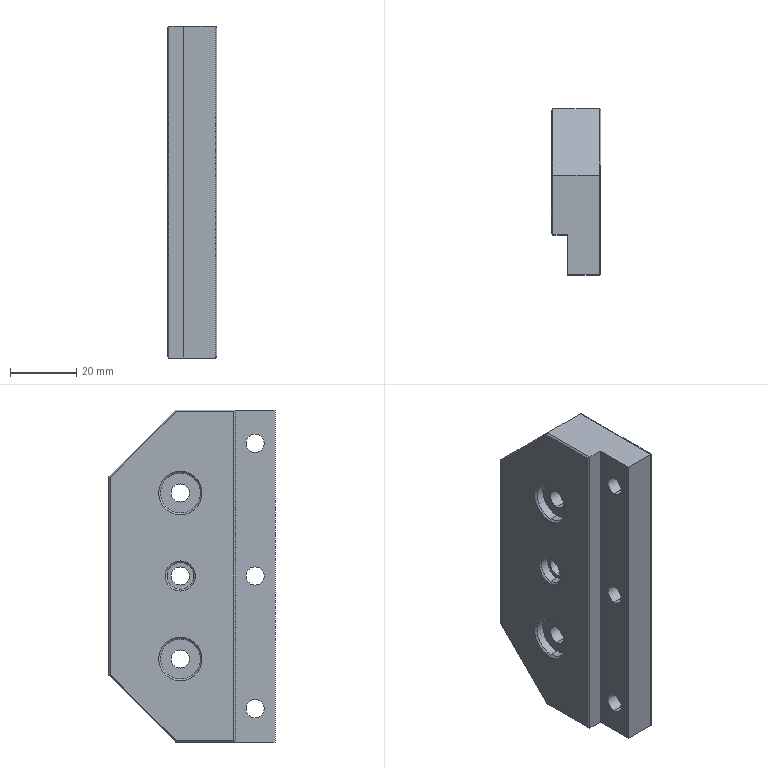Component | SolidWorks | Z-AxisElectricScrewdriverFixingPlateTopPlate-1 | 1 solid | 79 faces | volume 58386 mm3 | cylinder 36 | plane 25 | torus 12 | cone 6 | commonest cylinder face diameters 10 x12 5.5 x12 1 x6 12.1 x4 8.1 x2